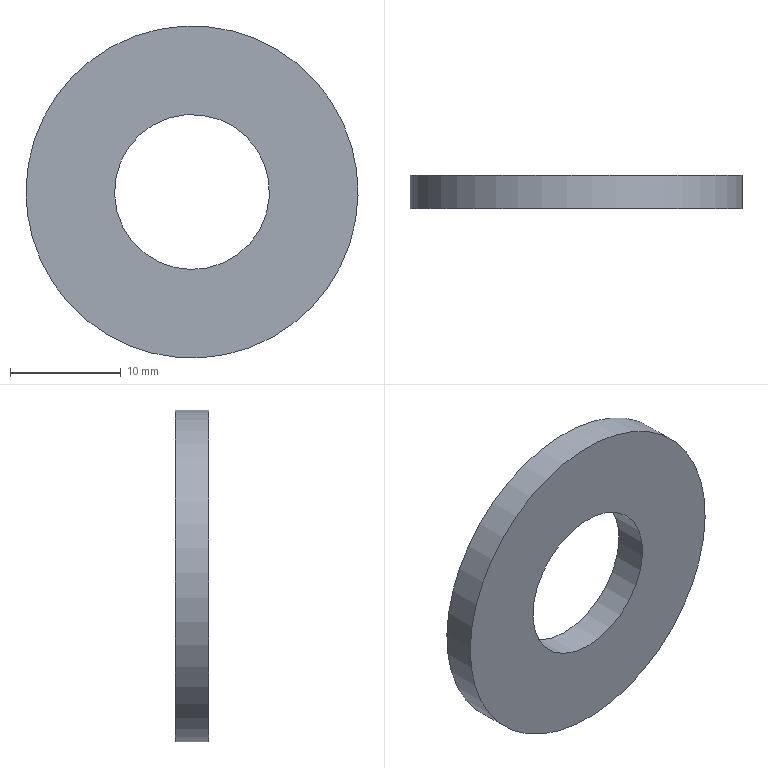Component | NX | WASHER | 1 solid | 4 faces | box 30 x 3 x 30 mm | volume 1659 mm3 | cylinder 2 | plane 2 | commonest cylinder face diameters 30 x1 14 x1
STEP:
#1=CARTESIAN_POINT('',(0.,0.,0.));
#2=DIRECTION('',(0.,0.,1.));
#3=DIRECTION('',(1.,0.,0.));
#4=AXIS2_PLACEMENT_3D('',#1,#2,#3);
#5=CARTESIAN_POINT('',(12.558,41.,51.204));
#6=VERTEX_POINT('',#5);
#7=CARTESIAN_POINT('',(-0.,41.,43.));
#8=DIRECTION('',(0.,-1.,0.));
#9=DIRECTION('',(0.8372,0.,0.5469));
#10=AXIS2_PLACEMENT_3D('',#7,#8,#9);
#11=CIRCLE('',#10,15.);
#12=CARTESIAN_POINT('',(-0.,41.,43.));
#13=DIRECTION('',(0.,1.,0.));
#14=DIRECTION('',(-0.8372,0.,-0.5469));
#15=AXIS2_PLACEMENT_3D('',#12,#13,#14);
#16=CYLINDRICAL_SURFACE('',#15,15.);
#17=CARTESIAN_POINT('',(9.425,0.));
#18=DIRECTION('',(-1.,0.));
#19=VECTOR('',#18,1.);
#20=LINE('',#17,#19);
#21=(GEOMETRIC_REPRESENTATION_CONTEXT(2)PARAMETRIC_REPRESENTATION_CONTEXT()REPRESENTATION_CONTEXT('',''));
#22=DEFINITIONAL_REPRESENTATION('',(#20),#21);
#23=PCURVE('',#16,#22);
#24=CARTESIAN_POINT('',(-0.,41.,43.));
#25=DIRECTION('',(0.,-1.,0.));
#26=DIRECTION('',(0.8372,0.,0.5469));
#27=AXIS2_PLACEMENT_3D('',#24,#25,#26);
#28=PLANE('',#27);
#29=CARTESIAN_POINT('',(0.,0.));
#30=DIRECTION('',(1.,0.));
#31=AXIS2_PLACEMENT_2D('',#29,#30);
#32=CIRCLE('',#31,15.);
#33=(GEOMETRIC_REPRESENTATION_CONTEXT(2)PARAMETRIC_REPRESENTATION_CONTEXT()REPRESENTATION_CONTEXT('',''));
#34=DEFINITIONAL_REPRESENTATION('',(#32),#33);
#35=PCURVE('',#28,#34);
#36=SURFACE_CURVE('',#11,(#23,#35),.PCURVE_S1.);
#37=EDGE_CURVE('',#6,#6,#36,.T.);
#38=ORIENTED_EDGE('',*,*,#37,.F.);
#39=CARTESIAN_POINT('',(12.558,44.,51.204));
#40=VERTEX_POINT('',#39);
#41=CARTESIAN_POINT('',(12.558,41.,51.204));
#42=CARTESIAN_POINT('',(12.558,44.,51.204));
#43=B_SPLINE_CURVE_WITH_KNOTS('',1,(#41,#42),.UNSPECIFIED.,.F.,.F.,(2,2),(0.,3.),.PIECEWISE_BEZIER_KNOTS.);
#44=CARTESIAN_POINT('',(9.425,0.));
#45=DIRECTION('',(0.,1.));
#46=VECTOR('',#45,1.);
#47=LINE('',#44,#46);
#48=(GEOMETRIC_REPRESENTATION_CONTEXT(2)PARAMETRIC_REPRESENTATION_CONTEXT()REPRESENTATION_CONTEXT('',''));
#49=DEFINITIONAL_REPRESENTATION('',(#47),#48);
#50=PCURVE('',#16,#49);
#51=CARTESIAN_POINT('',(3.142,0.));
#52=DIRECTION('',(0.,1.));
#53=VECTOR('',#52,1.);
#54=LINE('',#51,#53);
#55=(GEOMETRIC_REPRESENTATION_CONTEXT(2)PARAMETRIC_REPRESENTATION_CONTEXT()REPRESENTATION_CONTEXT('',''));
#56=DEFINITIONAL_REPRESENTATION('',(#54),#55);
#57=PCURVE('',#16,#56);
#58=SEAM_CURVE('',#43,(#50,#57),.PCURVE_S1.);
#59=EDGE_CURVE('',#6,#40,#58,.T.);
#60=ORIENTED_EDGE('',*,*,#59,.T.);
#61=CARTESIAN_POINT('',(-0.,44.,43.));
#62=DIRECTION('',(0.,-1.,0.));
#63=DIRECTION('',(0.8372,0.,0.5469));
#64=AXIS2_PLACEMENT_3D('',#61,#62,#63);
#65=CIRCLE('',#64,15.);
#66=CARTESIAN_POINT('',(9.425,3.));
#67=DIRECTION('',(-1.,0.));
#68=VECTOR('',#67,1.);
#69=LINE('',#66,#68);
#70=(GEOMETRIC_REPRESENTATION_CONTEXT(2)PARAMETRIC_REPRESENTATION_CONTEXT()REPRESENTATION_CONTEXT('',''));
#71=DEFINITIONAL_REPRESENTATION('',(#69),#70);
#72=PCURVE('',#16,#71);
#73=CARTESIAN_POINT('',(-0.,44.,43.));
#74=DIRECTION('',(0.,-1.,0.));
#75=DIRECTION('',(0.8372,0.,0.5469));
#76=AXIS2_PLACEMENT_3D('',#73,#74,#75);
#77=PLANE('',#76);
#78=CARTESIAN_POINT('',(0.,0.));
#79=DIRECTION('',(1.,0.));
#80=AXIS2_PLACEMENT_2D('',#78,#79);
#81=CIRCLE('',#80,15.);
#82=(GEOMETRIC_REPRESENTATION_CONTEXT(2)PARAMETRIC_REPRESENTATION_CONTEXT()REPRESENTATION_CONTEXT('',''));
#83=DEFINITIONAL_REPRESENTATION('',(#81),#82);
#84=PCURVE('',#77,#83);
#85=SURFACE_CURVE('',#65,(#72,#84),.PCURVE_S1.);
#86=EDGE_CURVE('',#40,#40,#85,.T.);
#87=ORIENTED_EDGE('',*,*,#86,.T.);
#88=ORIENTED_EDGE('',*,*,#59,.F.);
#89=EDGE_LOOP('',(#38,#60,#87,#88));
#90=FACE_BOUND('',#89,.T.);
#91=ADVANCED_FACE('',(#90),#16,.T.);
#92=CARTESIAN_POINT('',(5.86,41.,46.829));
#93=VERTEX_POINT('',#92);
#94=CARTESIAN_POINT('',(-0.,41.,43.));
#95=DIRECTION('',(0.,-1.,0.));
#96=DIRECTION('',(0.8372,0.,0.5469));
#97=AXIS2_PLACEMENT_3D('',#94,#95,#96);
#98=CIRCLE('',#97,7.);
#99=CARTESIAN_POINT('',(-0.,41.,43.));
#100=DIRECTION('',(0.,1.,0.));
#101=DIRECTION('',(-0.8372,0.,-0.5469));
#102=AXIS2_PLACEMENT_3D('',#99,#100,#101);
#103=CYLINDRICAL_SURFACE('',#102,7.);
#104=CARTESIAN_POINT('',(9.425,0.));
#105=DIRECTION('',(-1.,0.));
#106=VECTOR('',#105,1.);
#107=LINE('',#104,#106);
#108=(GEOMETRIC_REPRESENTATION_CONTEXT(2)PARAMETRIC_REPRESENTATION_CONTEXT()REPRESENTATION_CONTEXT('',''));
#109=DEFINITIONAL_REPRESENTATION('',(#107),#108);
#110=PCURVE('',#103,#109);
#111=CARTESIAN_POINT('',(0.,0.));
#112=DIRECTION('',(1.,0.));
#113=AXIS2_PLACEMENT_2D('',#111,#112);
#114=CIRCLE('',#113,7.);
#115=(GEOMETRIC_REPRESENTATION_CONTEXT(2)PARAMETRIC_REPRESENTATION_CONTEXT()REPRESENTATION_CONTEXT('',''));
#116=DEFINITIONAL_REPRESENTATION('',(#114),#115);
#117=PCURVE('',#28,#116);
#118=SURFACE_CURVE('',#98,(#110,#117),.PCURVE_S1.);
#119=EDGE_CURVE('',#93,#93,#118,.T.);
#120=ORIENTED_EDGE('',*,*,#119,.F.);
#121=CARTESIAN_POINT('',(5.86,44.,46.829));
#122=VERTEX_POINT('',#121);
#123=CARTESIAN_POINT('',(5.86,41.,46.829));
#124=CARTESIAN_POINT('',(5.86,44.,46.829));
#125=B_SPLINE_CURVE_WITH_KNOTS('',1,(#123,#124),.UNSPECIFIED.,.F.,.F.,(2,2),(0.,3.),.PIECEWISE_BEZIER_KNOTS.);
#126=CARTESIAN_POINT('',(9.425,0.));
#127=DIRECTION('',(0.,1.));
#128=VECTOR('',#127,1.);
#129=LINE('',#126,#128);
#130=(GEOMETRIC_REPRESENTATION_CONTEXT(2)PARAMETRIC_REPRESENTATION_CONTEXT()REPRESENTATION_CONTEXT('',''));
#131=DEFINITIONAL_REPRESENTATION('',(#129),#130);
#132=PCURVE('',#103,#131);
#133=CARTESIAN_POINT('',(3.142,0.));
#134=DIRECTION('',(0.,1.));
#135=VECTOR('',#134,1.);
#136=LINE('',#133,#135);
#137=(GEOMETRIC_REPRESENTATION_CONTEXT(2)PARAMETRIC_REPRESENTATION_CONTEXT()REPRESENTATION_CONTEXT('',''));
#138=DEFINITIONAL_REPRESENTATION('',(#136),#137);
#139=PCURVE('',#103,#138);
#140=SEAM_CURVE('',#125,(#132,#139),.PCURVE_S1.);
#141=EDGE_CURVE('',#93,#122,#140,.T.);
#142=ORIENTED_EDGE('',*,*,#141,.T.);
#143=CARTESIAN_POINT('',(-0.,44.,43.));
#144=DIRECTION('',(0.,-1.,0.));
#145=DIRECTION('',(0.8372,0.,0.5469));
#146=AXIS2_PLACEMENT_3D('',#143,#144,#145);
#147=CIRCLE('',#146,7.);
#148=CARTESIAN_POINT('',(9.425,3.));
#149=DIRECTION('',(-1.,0.));
#150=VECTOR('',#149,1.);
#151=LINE('',#148,#150);
#152=(GEOMETRIC_REPRESENTATION_CONTEXT(2)PARAMETRIC_REPRESENTATION_CONTEXT()REPRESENTATION_CONTEXT('',''));
#153=DEFINITIONAL_REPRESENTATION('',(#151),#152);
#154=PCURVE('',#103,#153);
#155=CARTESIAN_POINT('',(0.,0.));
#156=DIRECTION('',(1.,0.));
#157=AXIS2_PLACEMENT_2D('',#155,#156);
#158=CIRCLE('',#157,7.);
#159=(GEOMETRIC_REPRESENTATION_CONTEXT(2)PARAMETRIC_REPRESENTATION_CONTEXT()REPRESENTATION_CONTEXT('',''));
#160=DEFINITIONAL_REPRESENTATION('',(#158),#159);
#161=PCURVE('',#77,#160);
#162=SURFACE_CURVE('',#147,(#154,#161),.PCURVE_S1.);
#163=EDGE_CURVE('',#122,#122,#162,.T.);
#164=ORIENTED_EDGE('',*,*,#163,.T.);
#165=ORIENTED_EDGE('',*,*,#141,.F.);
#166=EDGE_LOOP('',(#120,#142,#164,#165));
#167=FACE_BOUND('',#166,.F.);
#168=ADVANCED_FACE('',(#167),#103,.F.);
#169=ORIENTED_EDGE('',*,*,#37,.T.);
#170=EDGE_LOOP('',(#169));
#171=FACE_BOUND('',#170,.T.);
#172=ORIENTED_EDGE('',*,*,#119,.F.);
#173=EDGE_LOOP('',(#172));
#174=FACE_BOUND('',#173,.T.);
#175=ADVANCED_FACE('',(#171,#174),#28,.T.);
#176=ORIENTED_EDGE('',*,*,#86,.F.);
#177=EDGE_LOOP('',(#176));
#178=FACE_BOUND('',#177,.T.);
#179=ORIENTED_EDGE('',*,*,#163,.T.);
#180=EDGE_LOOP('',(#179));
#181=FACE_BOUND('',#180,.T.);
#182=ADVANCED_FACE('',(#178,#181),#77,.F.);
#183=CLOSED_SHELL('',(#91,#168,#175,#182));
#184=MANIFOLD_SOLID_BREP('',#183);
#185=(LENGTH_UNIT()NAMED_UNIT(*)SI_UNIT(.MILLI.,.METRE.));
#186=UNCERTAINTY_MEASURE_WITH_UNIT(LENGTH_MEASURE(0.00001),#185,'','');
#187=(NAMED_UNIT(*)PLANE_ANGLE_UNIT()SI_UNIT($,.RADIAN.));
#188=(NAMED_UNIT(*)SI_UNIT($,.STERADIAN.)SOLID_ANGLE_UNIT());
#189=(GEOMETRIC_REPRESENTATION_CONTEXT(3)GLOBAL_UNCERTAINTY_ASSIGNED_CONTEXT((#186))GLOBAL_UNIT_ASSIGNED_CONTEXT((#185,#187,#188))REPRESENTATION_CONTEXT('',''));
#190=ADVANCED_BREP_SHAPE_REPRESENTATION('',(#4,#184),#189);